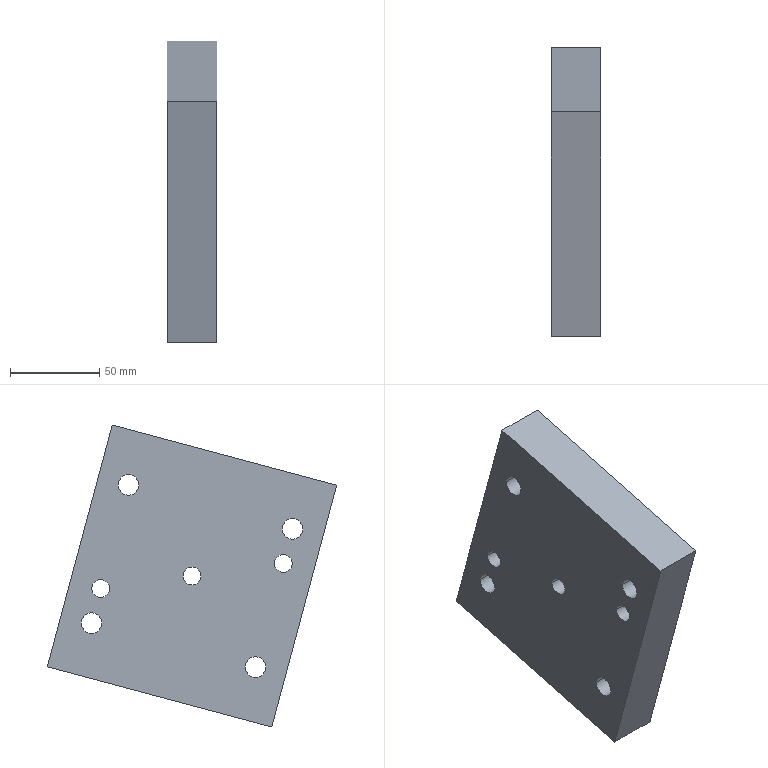Component | SolidWorks | EndFacePressurePlate-1 | 1 solid | 20 faces | box 27.78 x 161.81 x 168.88 mm | volume 487328 mm3 | cylinder 14 | plane 6 | commonest cylinder face diameters 11.57 x8 10 x6
build123d program:
from build123d import *

# Parameters (mm, degrees)
SKETCH1_R           = 5
SKETCH1_R_2         = 5.785
BOSS_EXTRUDE1_DEPTH = 27.778


with BuildPart() as part:
    # Sketch1 → Boss-Extrude1 (new body)
    with BuildSketch(Plane.XY.offset(27.778)):
        Polygon((197.028, -109.036), (71.458, -142.682), (107.693, -277.912), (233.263, -244.265), align=None)
        with Locations(Location((152.36, -193.474, 0), (0, 0, 180))):
            Circle(SKETCH1_R, mode=Mode.SUBTRACT)
        with Locations(Location((101.303, -186.449, 0), (0, 0, 180))):
            Circle(SKETCH1_R, mode=Mode.SUBTRACT)
        with Locations(Location((96.126, -167.131, 0), (0, 0, 180))):
            Circle(SKETCH1_R_2, mode=Mode.SUBTRACT)
        with Locations(Location((208.595, -219.817, 0), (0, 0, 180))):
            Circle(SKETCH1_R_2, mode=Mode.SUBTRACT)
        with Locations(Location((116.832, -244.405, 0), (0, 0, 180))):
            Circle(SKETCH1_R_2, mode=Mode.SUBTRACT)
        with Locations(Location((187.889, -142.543, 0), (0, 0, 180))):
            Circle(SKETCH1_R_2, mode=Mode.SUBTRACT)
        with Locations(Location((203.418, -200.498, 0), (0, 0, 180))):
            Circle(SKETCH1_R, mode=Mode.SUBTRACT)
    extrude(amount=-BOSS_EXTRUDE1_DEPTH)


solid = part.part

# Placed as in the assembly
solid = solid.moved(Location((-252.332, 870.769, 1116.347), (90, 90, 0)))
STEP:
#1=COLOUR_RGB('',0.7922,0.8196,0.9333);
#2=FILL_AREA_STYLE_COLOUR('',#1);
#3=FILL_AREA_STYLE('',(#2));
#4=SURFACE_STYLE_FILL_AREA(#3);
#5=SURFACE_SIDE_STYLE('',(#4));
#6=SURFACE_STYLE_USAGE(.BOTH.,#5);
#7=PRESENTATION_STYLE_ASSIGNMENT((#6));
#8=CARTESIAN_POINT('',(-9.934,42.094,36.057));
#9=VERTEX_POINT('',#8);
#10=CARTESIAN_POINT('',(-9.934,42.488,36.057));
#11=VERTEX_POINT('',#10);
#12=CARTESIAN_POINT('',(-9.934,42.291,36.057));
#13=DIRECTION('',(1.,0.,0.));
#14=DIRECTION('',(0.,-1.,0.));
#15=AXIS2_PLACEMENT_3D('',#12,#13,#14);
#16=CIRCLE('',#15,0.1969);
#17=EDGE_CURVE('',#9,#11,#16,.T.);
#18=ORIENTED_EDGE('',*,*,#17,.F.);
#19=CARTESIAN_POINT('',(-8.841,42.094,36.057));
#20=VERTEX_POINT('',#19);
#21=CARTESIAN_POINT('',(-9.934,42.094,36.057));
#22=DIRECTION('',(1.,0.,0.));
#23=VECTOR('',#22,39.37);
#24=LINE('',#21,#23);
#25=EDGE_CURVE('',#9,#20,#24,.T.);
#26=ORIENTED_EDGE('',*,*,#25,.T.);
#27=CARTESIAN_POINT('',(-8.841,42.488,36.057));
#28=VERTEX_POINT('',#27);
#29=CARTESIAN_POINT('',(-8.841,42.291,36.057));
#30=DIRECTION('',(1.,0.,0.));
#31=DIRECTION('',(0.,-1.,0.));
#32=AXIS2_PLACEMENT_3D('',#29,#30,#31);
#33=CIRCLE('',#32,0.1969);
#34=EDGE_CURVE('',#20,#28,#33,.T.);
#35=ORIENTED_EDGE('',*,*,#34,.T.);
#36=CARTESIAN_POINT('',(-9.934,42.488,36.057));
#37=DIRECTION('',(1.,0.,0.));
#38=VECTOR('',#37,39.37);
#39=LINE('',#36,#38);
#40=EDGE_CURVE('',#11,#28,#39,.T.);
#41=ORIENTED_EDGE('',*,*,#40,.F.);
#42=EDGE_LOOP('',(#18,#26,#35,#41));
#43=FACE_OUTER_BOUND('',#42,.T.);
#44=CARTESIAN_POINT('',(-9.934,42.291,36.057));
#45=DIRECTION('',(1.,0.,0.));
#46=DIRECTION('',(0.,1.,0.));
#47=AXIS2_PLACEMENT_3D('',#44,#45,#46);
#48=CYLINDRICAL_SURFACE('',#47,0.1969);
#49=ADVANCED_FACE('',(#43),#48,.F.);
#50=CARTESIAN_POINT('',(-9.934,41.452,38.339));
#51=VERTEX_POINT('',#50);
#52=CARTESIAN_POINT('',(-9.934,41.907,38.339));
#53=VERTEX_POINT('',#52);
#54=CARTESIAN_POINT('',(-9.934,41.679,38.339));
#55=DIRECTION('',(1.,0.,0.));
#56=DIRECTION('',(0.,-1.,0.));
#57=AXIS2_PLACEMENT_3D('',#54,#55,#56);
#58=CIRCLE('',#57,0.2278);
#59=EDGE_CURVE('',#51,#53,#58,.T.);
#60=ORIENTED_EDGE('',*,*,#59,.F.);
#61=CARTESIAN_POINT('',(-8.841,41.452,38.339));
#62=VERTEX_POINT('',#61);
#63=CARTESIAN_POINT('',(-9.934,41.452,38.339));
#64=DIRECTION('',(1.,0.,0.));
#65=VECTOR('',#64,39.37);
#66=LINE('',#63,#65);
#67=EDGE_CURVE('',#51,#62,#66,.T.);
#68=ORIENTED_EDGE('',*,*,#67,.T.);
#69=CARTESIAN_POINT('',(-8.841,41.907,38.339));
#70=VERTEX_POINT('',#69);
#71=CARTESIAN_POINT('',(-8.841,41.679,38.339));
#72=DIRECTION('',(1.,0.,0.));
#73=DIRECTION('',(0.,-1.,0.));
#74=AXIS2_PLACEMENT_3D('',#71,#72,#73);
#75=CIRCLE('',#74,0.2278);
#76=EDGE_CURVE('',#62,#70,#75,.T.);
#77=ORIENTED_EDGE('',*,*,#76,.T.);
#78=CARTESIAN_POINT('',(-9.934,41.907,38.339));
#79=DIRECTION('',(1.,0.,0.));
#80=VECTOR('',#79,39.37);
#81=LINE('',#78,#80);
#82=EDGE_CURVE('',#53,#70,#81,.T.);
#83=ORIENTED_EDGE('',*,*,#82,.F.);
#84=EDGE_LOOP('',(#60,#68,#77,#83));
#85=FACE_OUTER_BOUND('',#84,.T.);
#86=CARTESIAN_POINT('',(-9.934,41.679,38.339));
#87=DIRECTION('',(1.,0.,0.));
#88=DIRECTION('',(0.,1.,0.));
#89=AXIS2_PLACEMENT_3D('',#86,#87,#88);
#90=CYLINDRICAL_SURFACE('',#89,0.2278);
#91=ADVANCED_FACE('',(#85),#90,.F.);
#92=CARTESIAN_POINT('',(-9.934,38.654,34.328));
#93=VERTEX_POINT('',#92);
#94=CARTESIAN_POINT('',(-9.934,39.11,34.328));
#95=VERTEX_POINT('',#94);
#96=CARTESIAN_POINT('',(-9.934,38.882,34.328));
#97=DIRECTION('',(1.,0.,0.));
#98=DIRECTION('',(0.,-1.,0.));
#99=AXIS2_PLACEMENT_3D('',#96,#97,#98);
#100=CIRCLE('',#99,0.2278);
#101=EDGE_CURVE('',#93,#95,#100,.T.);
#102=ORIENTED_EDGE('',*,*,#101,.F.);
#103=CARTESIAN_POINT('',(-8.841,38.654,34.328));
#104=VERTEX_POINT('',#103);
#105=CARTESIAN_POINT('',(-9.934,38.654,34.328));
#106=DIRECTION('',(1.,0.,0.));
#107=VECTOR('',#106,39.37);
#108=LINE('',#105,#107);
#109=EDGE_CURVE('',#93,#104,#108,.T.);
#110=ORIENTED_EDGE('',*,*,#109,.T.);
#111=CARTESIAN_POINT('',(-8.841,39.11,34.328));
#112=VERTEX_POINT('',#111);
#113=CARTESIAN_POINT('',(-8.841,38.882,34.328));
#114=DIRECTION('',(1.,0.,0.));
#115=DIRECTION('',(0.,-1.,0.));
#116=AXIS2_PLACEMENT_3D('',#113,#114,#115);
#117=CIRCLE('',#116,0.2278);
#118=EDGE_CURVE('',#104,#112,#117,.T.);
#119=ORIENTED_EDGE('',*,*,#118,.T.);
#120=CARTESIAN_POINT('',(-9.934,39.11,34.328));
#121=DIRECTION('',(1.,0.,0.));
#122=VECTOR('',#121,39.37);
#123=LINE('',#120,#122);
#124=EDGE_CURVE('',#95,#112,#123,.T.);
#125=ORIENTED_EDGE('',*,*,#124,.F.);
#126=EDGE_LOOP('',(#102,#110,#119,#125));
#127=FACE_OUTER_BOUND('',#126,.T.);
#128=CARTESIAN_POINT('',(-9.934,38.882,34.328));
#129=DIRECTION('',(1.,0.,0.));
#130=DIRECTION('',(0.,1.,0.));
#131=AXIS2_PLACEMENT_3D('',#128,#129,#130);
#132=CYLINDRICAL_SURFACE('',#131,0.2278);
#133=ADVANCED_FACE('',(#127),#132,.F.);
#134=CARTESIAN_POINT('',(-9.934,42.267,35.296));
#135=VERTEX_POINT('',#134);
#136=CARTESIAN_POINT('',(-9.934,42.722,35.296));
#137=VERTEX_POINT('',#136);
#138=CARTESIAN_POINT('',(-9.934,42.495,35.296));
#139=DIRECTION('',(1.,0.,0.));
#140=DIRECTION('',(0.,-1.,0.));
#141=AXIS2_PLACEMENT_3D('',#138,#139,#140);
#142=CIRCLE('',#141,0.2278);
#143=EDGE_CURVE('',#135,#137,#142,.T.);
#144=ORIENTED_EDGE('',*,*,#143,.F.);
#145=CARTESIAN_POINT('',(-8.841,42.267,35.296));
#146=VERTEX_POINT('',#145);
#147=CARTESIAN_POINT('',(-9.934,42.267,35.296));
#148=DIRECTION('',(1.,0.,0.));
#149=VECTOR('',#148,39.37);
#150=LINE('',#147,#149);
#151=EDGE_CURVE('',#135,#146,#150,.T.);
#152=ORIENTED_EDGE('',*,*,#151,.T.);
#153=CARTESIAN_POINT('',(-8.841,42.722,35.296));
#154=VERTEX_POINT('',#153);
#155=CARTESIAN_POINT('',(-8.841,42.495,35.296));
#156=DIRECTION('',(1.,0.,0.));
#157=DIRECTION('',(0.,-1.,0.));
#158=AXIS2_PLACEMENT_3D('',#155,#156,#157);
#159=CIRCLE('',#158,0.2278);
#160=EDGE_CURVE('',#146,#154,#159,.T.);
#161=ORIENTED_EDGE('',*,*,#160,.T.);
#162=CARTESIAN_POINT('',(-9.934,42.722,35.296));
#163=DIRECTION('',(1.,0.,0.));
#164=VECTOR('',#163,39.37);
#165=LINE('',#162,#164);
#166=EDGE_CURVE('',#137,#154,#165,.T.);
#167=ORIENTED_EDGE('',*,*,#166,.F.);
#168=EDGE_LOOP('',(#144,#152,#161,#167));
#169=FACE_OUTER_BOUND('',#168,.T.);
#170=CARTESIAN_POINT('',(-9.934,42.495,35.296));
#171=DIRECTION('',(1.,0.,0.));
#172=DIRECTION('',(0.,1.,0.));
#173=AXIS2_PLACEMENT_3D('',#170,#171,#172);
#174=CYLINDRICAL_SURFACE('',#173,0.2278);
#175=ADVANCED_FACE('',(#169),#174,.F.);
#176=CARTESIAN_POINT('',(-9.934,37.839,37.371));
#177=VERTEX_POINT('',#176);
#178=CARTESIAN_POINT('',(-9.934,38.294,37.371));
#179=VERTEX_POINT('',#178);
#180=CARTESIAN_POINT('',(-9.934,38.067,37.371));
#181=DIRECTION('',(1.,0.,0.));
#182=DIRECTION('',(0.,-1.,0.));
#183=AXIS2_PLACEMENT_3D('',#180,#181,#182);
#184=CIRCLE('',#183,0.2278);
#185=EDGE_CURVE('',#177,#179,#184,.T.);
#186=ORIENTED_EDGE('',*,*,#185,.F.);
#187=CARTESIAN_POINT('',(-8.841,37.839,37.371));
#188=VERTEX_POINT('',#187);
#189=CARTESIAN_POINT('',(-9.934,37.839,37.371));
#190=DIRECTION('',(1.,0.,0.));
#191=VECTOR('',#190,39.37);
#192=LINE('',#189,#191);
#193=EDGE_CURVE('',#177,#188,#192,.T.);
#194=ORIENTED_EDGE('',*,*,#193,.T.);
#195=CARTESIAN_POINT('',(-8.841,38.294,37.371));
#196=VERTEX_POINT('',#195);
#197=CARTESIAN_POINT('',(-8.841,38.067,37.371));
#198=DIRECTION('',(1.,0.,0.));
#199=DIRECTION('',(0.,-1.,0.));
#200=AXIS2_PLACEMENT_3D('',#197,#198,#199);
#201=CIRCLE('',#200,0.2278);
#202=EDGE_CURVE('',#188,#196,#201,.T.);
#203=ORIENTED_EDGE('',*,*,#202,.T.);
#204=CARTESIAN_POINT('',(-9.934,38.294,37.371));
#205=DIRECTION('',(1.,0.,0.));
#206=VECTOR('',#205,39.37);
#207=LINE('',#204,#206);
#208=EDGE_CURVE('',#179,#196,#207,.T.);
#209=ORIENTED_EDGE('',*,*,#208,.F.);
#210=EDGE_LOOP('',(#186,#194,#203,#209));
#211=FACE_OUTER_BOUND('',#210,.T.);
#212=CARTESIAN_POINT('',(-9.934,38.067,37.371));
#213=DIRECTION('',(1.,0.,0.));
#214=DIRECTION('',(0.,1.,0.));
#215=AXIS2_PLACEMENT_3D('',#212,#213,#214);
#216=CYLINDRICAL_SURFACE('',#215,0.2278);
#217=ADVANCED_FACE('',(#211),#216,.F.);
#218=CARTESIAN_POINT('',(-9.934,38.074,36.61));
#219=VERTEX_POINT('',#218);
#220=CARTESIAN_POINT('',(-9.934,38.467,36.61));
#221=VERTEX_POINT('',#220);
#222=CARTESIAN_POINT('',(-9.934,38.271,36.61));
#223=DIRECTION('',(1.,0.,0.));
#224=DIRECTION('',(0.,-1.,0.));
#225=AXIS2_PLACEMENT_3D('',#222,#223,#224);
#226=CIRCLE('',#225,0.1969);
#227=EDGE_CURVE('',#219,#221,#226,.T.);
#228=ORIENTED_EDGE('',*,*,#227,.F.);
#229=CARTESIAN_POINT('',(-8.841,38.074,36.61));
#230=VERTEX_POINT('',#229);
#231=CARTESIAN_POINT('',(-9.934,38.074,36.61));
#232=DIRECTION('',(1.,0.,0.));
#233=VECTOR('',#232,39.37);
#234=LINE('',#231,#233);
#235=EDGE_CURVE('',#219,#230,#234,.T.);
#236=ORIENTED_EDGE('',*,*,#235,.T.);
#237=CARTESIAN_POINT('',(-8.841,38.467,36.61));
#238=VERTEX_POINT('',#237);
#239=CARTESIAN_POINT('',(-8.841,38.271,36.61));
#240=DIRECTION('',(1.,0.,0.));
#241=DIRECTION('',(0.,-1.,0.));
#242=AXIS2_PLACEMENT_3D('',#239,#240,#241);
#243=CIRCLE('',#242,0.1969);
#244=EDGE_CURVE('',#230,#238,#243,.T.);
#245=ORIENTED_EDGE('',*,*,#244,.T.);
#246=CARTESIAN_POINT('',(-9.934,38.467,36.61));
#247=DIRECTION('',(1.,0.,0.));
#248=VECTOR('',#247,39.37);
#249=LINE('',#246,#248);
#250=EDGE_CURVE('',#221,#238,#249,.T.);
#251=ORIENTED_EDGE('',*,*,#250,.F.);
#252=EDGE_LOOP('',(#228,#236,#245,#251));
#253=FACE_OUTER_BOUND('',#252,.T.);
#254=CARTESIAN_POINT('',(-9.934,38.271,36.61));
#255=DIRECTION('',(1.,0.,0.));
#256=DIRECTION('',(0.,1.,0.));
#257=AXIS2_PLACEMENT_3D('',#254,#255,#256);
#258=CYLINDRICAL_SURFACE('',#257,0.1969);
#259=ADVANCED_FACE('',(#253),#258,.F.);
#260=CARTESIAN_POINT('',(-9.934,40.084,36.334));
#261=VERTEX_POINT('',#260);
#262=CARTESIAN_POINT('',(-9.934,40.478,36.334));
#263=VERTEX_POINT('',#262);
#264=CARTESIAN_POINT('',(-9.934,40.281,36.334));
#265=DIRECTION('',(1.,0.,0.));
#266=DIRECTION('',(0.,-1.,0.));
#267=AXIS2_PLACEMENT_3D('',#264,#265,#266);
#268=CIRCLE('',#267,0.1969);
#269=EDGE_CURVE('',#261,#263,#268,.T.);
#270=ORIENTED_EDGE('',*,*,#269,.F.);
#271=CARTESIAN_POINT('',(-8.841,40.084,36.334));
#272=VERTEX_POINT('',#271);
#273=CARTESIAN_POINT('',(-9.934,40.084,36.334));
#274=DIRECTION('',(1.,0.,0.));
#275=VECTOR('',#274,39.37);
#276=LINE('',#273,#275);
#277=EDGE_CURVE('',#261,#272,#276,.T.);
#278=ORIENTED_EDGE('',*,*,#277,.T.);
#279=CARTESIAN_POINT('',(-8.841,40.478,36.334));
#280=VERTEX_POINT('',#279);
#281=CARTESIAN_POINT('',(-8.841,40.281,36.334));
#282=DIRECTION('',(1.,0.,0.));
#283=DIRECTION('',(0.,-1.,0.));
#284=AXIS2_PLACEMENT_3D('',#281,#282,#283);
#285=CIRCLE('',#284,0.1969);
#286=EDGE_CURVE('',#272,#280,#285,.T.);
#287=ORIENTED_EDGE('',*,*,#286,.T.);
#288=CARTESIAN_POINT('',(-9.934,40.478,36.334));
#289=DIRECTION('',(1.,0.,0.));
#290=VECTOR('',#289,39.37);
#291=LINE('',#288,#290);
#292=EDGE_CURVE('',#263,#280,#291,.T.);
#293=ORIENTED_EDGE('',*,*,#292,.F.);
#294=EDGE_LOOP('',(#270,#278,#287,#293));
#295=FACE_OUTER_BOUND('',#294,.T.);
#296=CARTESIAN_POINT('',(-9.934,40.281,36.334));
#297=DIRECTION('',(1.,0.,0.));
#298=DIRECTION('',(0.,1.,0.));
#299=AXIS2_PLACEMENT_3D('',#296,#297,#298);
#300=CYLINDRICAL_SURFACE('',#299,0.1969);
#301=ADVANCED_FACE('',(#295),#300,.F.);
#302=CARTESIAN_POINT('',(-8.841,43.466,34.334));
#303=VERTEX_POINT('',#302);
#304=CARTESIAN_POINT('',(-8.841,42.039,39.658));
#305=VERTEX_POINT('',#304);
#306=CARTESIAN_POINT('',(-8.841,43.466,34.334));
#307=DIRECTION('',(0.,-0.2588,0.9659));
#308=VECTOR('',#307,39.37);
#309=LINE('',#306,#308);
#310=EDGE_CURVE('',#303,#305,#309,.T.);
#311=ORIENTED_EDGE('',*,*,#310,.F.);
#312=CARTESIAN_POINT('',(-9.934,43.466,34.334));
#313=VERTEX_POINT('',#312);
#314=CARTESIAN_POINT('',(-9.934,43.466,34.334));
#315=DIRECTION('',(1.,0.,0.));
#316=VECTOR('',#315,39.37);
#317=LINE('',#314,#316);
#318=EDGE_CURVE('',#313,#303,#317,.T.);
#319=ORIENTED_EDGE('',*,*,#318,.F.);
#320=CARTESIAN_POINT('',(-9.934,42.039,39.658));
#321=VERTEX_POINT('',#320);
#322=CARTESIAN_POINT('',(-9.934,43.466,34.334));
#323=DIRECTION('',(0.,-0.2588,0.9659));
#324=VECTOR('',#323,39.37);
#325=LINE('',#322,#324);
#326=EDGE_CURVE('',#313,#321,#325,.T.);
#327=ORIENTED_EDGE('',*,*,#326,.T.);
#328=CARTESIAN_POINT('',(-9.934,42.039,39.658));
#329=DIRECTION('',(1.,0.,0.));
#330=VECTOR('',#329,39.37);
#331=LINE('',#328,#330);
#332=EDGE_CURVE('',#321,#305,#331,.T.);
#333=ORIENTED_EDGE('',*,*,#332,.T.);
#334=EDGE_LOOP('',(#311,#319,#327,#333));
#335=FACE_OUTER_BOUND('',#334,.T.);
#336=CARTESIAN_POINT('',(-9.934,43.466,34.334));
#337=DIRECTION('',(0.,0.9659,0.2588));
#338=DIRECTION('',(0.,-0.2588,0.9659));
#339=AXIS2_PLACEMENT_3D('',#336,#337,#338);
#340=PLANE('',#339);
#341=ADVANCED_FACE('',(#335),#340,.T.);
#342=CARTESIAN_POINT('',(-8.841,38.522,33.009));
#343=VERTEX_POINT('',#342);
#344=CARTESIAN_POINT('',(-8.841,38.522,33.009));
#345=DIRECTION('',(0.,0.9659,0.2588));
#346=VECTOR('',#345,39.37);
#347=LINE('',#344,#346);
#348=EDGE_CURVE('',#343,#303,#347,.T.);
#349=ORIENTED_EDGE('',*,*,#348,.F.);
#350=CARTESIAN_POINT('',(-9.934,38.522,33.009));
#351=VERTEX_POINT('',#350);
#352=CARTESIAN_POINT('',(-9.934,38.522,33.009));
#353=DIRECTION('',(1.,0.,0.));
#354=VECTOR('',#353,39.37);
#355=LINE('',#352,#354);
#356=EDGE_CURVE('',#351,#343,#355,.T.);
#357=ORIENTED_EDGE('',*,*,#356,.F.);
#358=CARTESIAN_POINT('',(-9.934,38.522,33.009));
#359=DIRECTION('',(0.,0.9659,0.2588));
#360=VECTOR('',#359,39.37);
#361=LINE('',#358,#360);
#362=EDGE_CURVE('',#351,#313,#361,.T.);
#363=ORIENTED_EDGE('',*,*,#362,.T.);
#364=ORIENTED_EDGE('',*,*,#318,.T.);
#365=EDGE_LOOP('',(#349,#357,#363,#364));
#366=FACE_OUTER_BOUND('',#365,.T.);
#367=CARTESIAN_POINT('',(-9.934,38.522,33.009));
#368=DIRECTION('',(0.,0.2588,-0.9659));
#369=DIRECTION('',(0.,0.9659,0.2588));
#370=AXIS2_PLACEMENT_3D('',#367,#368,#369);
#371=PLANE('',#370);
#372=ADVANCED_FACE('',(#366),#371,.T.);
#373=CARTESIAN_POINT('',(-8.841,37.096,38.333));
#374=VERTEX_POINT('',#373);
#375=CARTESIAN_POINT('',(-8.841,37.096,38.333));
#376=DIRECTION('',(0.,0.2588,-0.9659));
#377=VECTOR('',#376,39.37);
#378=LINE('',#375,#377);
#379=EDGE_CURVE('',#374,#343,#378,.T.);
#380=ORIENTED_EDGE('',*,*,#379,.F.);
#381=CARTESIAN_POINT('',(-9.934,37.096,38.333));
#382=VERTEX_POINT('',#381);
#383=CARTESIAN_POINT('',(-9.934,37.096,38.333));
#384=DIRECTION('',(1.,0.,0.));
#385=VECTOR('',#384,39.37);
#386=LINE('',#383,#385);
#387=EDGE_CURVE('',#382,#374,#386,.T.);
#388=ORIENTED_EDGE('',*,*,#387,.F.);
#389=CARTESIAN_POINT('',(-9.934,37.096,38.333));
#390=DIRECTION('',(0.,0.2588,-0.9659));
#391=VECTOR('',#390,39.37);
#392=LINE('',#389,#391);
#393=EDGE_CURVE('',#382,#351,#392,.T.);
#394=ORIENTED_EDGE('',*,*,#393,.T.);
#395=ORIENTED_EDGE('',*,*,#356,.T.);
#396=EDGE_LOOP('',(#380,#388,#394,#395));
#397=FACE_OUTER_BOUND('',#396,.T.);
#398=CARTESIAN_POINT('',(-9.934,37.096,38.333));
#399=DIRECTION('',(0.,-0.9659,-0.2588));
#400=DIRECTION('',(0.,0.2588,-0.9659));
#401=AXIS2_PLACEMENT_3D('',#398,#399,#400);
#402=PLANE('',#401);
#403=ADVANCED_FACE('',(#397),#402,.T.);
#404=CARTESIAN_POINT('',(-8.841,42.039,39.658));
#405=DIRECTION('',(0.,-0.9659,-0.2588));
#406=VECTOR('',#405,39.37);
#407=LINE('',#404,#406);
#408=EDGE_CURVE('',#305,#374,#407,.T.);
#409=ORIENTED_EDGE('',*,*,#408,.F.);
#410=ORIENTED_EDGE('',*,*,#332,.F.);
#411=CARTESIAN_POINT('',(-9.934,42.039,39.658));
#412=DIRECTION('',(0.,-0.9659,-0.2588));
#413=VECTOR('',#412,39.37);
#414=LINE('',#411,#413);
#415=EDGE_CURVE('',#321,#382,#414,.T.);
#416=ORIENTED_EDGE('',*,*,#415,.T.);
#417=ORIENTED_EDGE('',*,*,#387,.T.);
#418=EDGE_LOOP('',(#409,#410,#416,#417));
#419=FACE_OUTER_BOUND('',#418,.T.);
#420=CARTESIAN_POINT('',(-9.934,42.039,39.658));
#421=DIRECTION('',(0.,-0.2588,0.9659));
#422=DIRECTION('',(0.,-0.9659,-0.2588));
#423=AXIS2_PLACEMENT_3D('',#420,#421,#422);
#424=PLANE('',#423);
#425=ADVANCED_FACE('',(#419),#424,.T.);
#426=CARTESIAN_POINT('',(-9.934,42.291,36.057));
#427=DIRECTION('',(1.,0.,0.));
#428=DIRECTION('',(0.,-1.,0.));
#429=AXIS2_PLACEMENT_3D('',#426,#427,#428);
#430=CIRCLE('',#429,0.1969);
#431=EDGE_CURVE('',#11,#9,#430,.T.);
#432=ORIENTED_EDGE('',*,*,#431,.T.);
#433=ORIENTED_EDGE('',*,*,#17,.T.);
#434=EDGE_LOOP('',(#432,#433));
#435=FACE_BOUND('',#434,.T.);
#436=CARTESIAN_POINT('',(-9.934,41.679,38.339));
#437=DIRECTION('',(1.,0.,0.));
#438=DIRECTION('',(0.,-1.,0.));
#439=AXIS2_PLACEMENT_3D('',#436,#437,#438);
#440=CIRCLE('',#439,0.2278);
#441=EDGE_CURVE('',#53,#51,#440,.T.);
#442=ORIENTED_EDGE('',*,*,#441,.T.);
#443=ORIENTED_EDGE('',*,*,#59,.T.);
#444=EDGE_LOOP('',(#442,#443));
#445=FACE_BOUND('',#444,.T.);
#446=CARTESIAN_POINT('',(-9.934,38.882,34.328));
#447=DIRECTION('',(1.,0.,0.));
#448=DIRECTION('',(0.,-1.,0.));
#449=AXIS2_PLACEMENT_3D('',#446,#447,#448);
#450=CIRCLE('',#449,0.2278);
#451=EDGE_CURVE('',#95,#93,#450,.T.);
#452=ORIENTED_EDGE('',*,*,#451,.T.);
#453=ORIENTED_EDGE('',*,*,#101,.T.);
#454=EDGE_LOOP('',(#452,#453));
#455=FACE_BOUND('',#454,.T.);
#456=CARTESIAN_POINT('',(-9.934,42.495,35.296));
#457=DIRECTION('',(1.,0.,0.));
#458=DIRECTION('',(0.,-1.,0.));
#459=AXIS2_PLACEMENT_3D('',#456,#457,#458);
#460=CIRCLE('',#459,0.2278);
#461=EDGE_CURVE('',#137,#135,#460,.T.);
#462=ORIENTED_EDGE('',*,*,#461,.T.);
#463=ORIENTED_EDGE('',*,*,#143,.T.);
#464=EDGE_LOOP('',(#462,#463));
#465=FACE_BOUND('',#464,.T.);
#466=CARTESIAN_POINT('',(-9.934,38.067,37.371));
#467=DIRECTION('',(1.,0.,0.));
#468=DIRECTION('',(0.,-1.,0.));
#469=AXIS2_PLACEMENT_3D('',#466,#467,#468);
#470=CIRCLE('',#469,0.2278);
#471=EDGE_CURVE('',#179,#177,#470,.T.);
#472=ORIENTED_EDGE('',*,*,#471,.T.);
#473=ORIENTED_EDGE('',*,*,#185,.T.);
#474=EDGE_LOOP('',(#472,#473));
#475=FACE_BOUND('',#474,.T.);
#476=CARTESIAN_POINT('',(-9.934,38.271,36.61));
#477=DIRECTION('',(1.,0.,0.));
#478=DIRECTION('',(0.,-1.,0.));
#479=AXIS2_PLACEMENT_3D('',#476,#477,#478);
#480=CIRCLE('',#479,0.1969);
#481=EDGE_CURVE('',#221,#219,#480,.T.);
#482=ORIENTED_EDGE('',*,*,#481,.T.);
#483=ORIENTED_EDGE('',*,*,#227,.T.);
#484=EDGE_LOOP('',(#482,#483));
#485=FACE_BOUND('',#484,.T.);
#486=CARTESIAN_POINT('',(-9.934,40.281,36.334));
#487=DIRECTION('',(1.,0.,0.));
#488=DIRECTION('',(0.,-1.,0.));
#489=AXIS2_PLACEMENT_3D('',#486,#487,#488);
#490=CIRCLE('',#489,0.1969);
#491=EDGE_CURVE('',#263,#261,#490,.T.);
#492=ORIENTED_EDGE('',*,*,#491,.T.);
#493=ORIENTED_EDGE('',*,*,#269,.T.);
#494=EDGE_LOOP('',(#492,#493));
#495=FACE_BOUND('',#494,.T.);
#496=ORIENTED_EDGE('',*,*,#326,.F.);
#497=ORIENTED_EDGE('',*,*,#362,.F.);
#498=ORIENTED_EDGE('',*,*,#393,.F.);
#499=ORIENTED_EDGE('',*,*,#415,.F.);
#500=EDGE_LOOP('',(#496,#497,#498,#499));
#501=FACE_OUTER_BOUND('',#500,.T.);
#502=CARTESIAN_POINT('',(-9.934,34.282,43.951));
#503=DIRECTION('',(1.,0.,0.));
#504=DIRECTION('',(0.,1.,0.));
#505=AXIS2_PLACEMENT_3D('',#502,#503,#504);
#506=PLANE('',#505);
#507=ADVANCED_FACE('',(#435,#445,#455,#465,#475,#485,#495,#501),#506,.F.);
#508=CARTESIAN_POINT('',(-8.841,42.291,36.057));
#509=DIRECTION('',(1.,0.,0.));
#510=DIRECTION('',(0.,-1.,0.));
#511=AXIS2_PLACEMENT_3D('',#508,#509,#510);
#512=CIRCLE('',#511,0.1969);
#513=EDGE_CURVE('',#28,#20,#512,.T.);
#514=ORIENTED_EDGE('',*,*,#513,.F.);
#515=ORIENTED_EDGE('',*,*,#34,.F.);
#516=EDGE_LOOP('',(#514,#515));
#517=FACE_BOUND('',#516,.T.);
#518=CARTESIAN_POINT('',(-8.841,41.679,38.339));
#519=DIRECTION('',(1.,0.,0.));
#520=DIRECTION('',(0.,-1.,0.));
#521=AXIS2_PLACEMENT_3D('',#518,#519,#520);
#522=CIRCLE('',#521,0.2278);
#523=EDGE_CURVE('',#70,#62,#522,.T.);
#524=ORIENTED_EDGE('',*,*,#523,.F.);
#525=ORIENTED_EDGE('',*,*,#76,.F.);
#526=EDGE_LOOP('',(#524,#525));
#527=FACE_BOUND('',#526,.T.);
#528=CARTESIAN_POINT('',(-8.841,38.882,34.328));
#529=DIRECTION('',(1.,0.,0.));
#530=DIRECTION('',(0.,-1.,0.));
#531=AXIS2_PLACEMENT_3D('',#528,#529,#530);
#532=CIRCLE('',#531,0.2278);
#533=EDGE_CURVE('',#112,#104,#532,.T.);
#534=ORIENTED_EDGE('',*,*,#533,.F.);
#535=ORIENTED_EDGE('',*,*,#118,.F.);
#536=EDGE_LOOP('',(#534,#535));
#537=FACE_BOUND('',#536,.T.);
#538=CARTESIAN_POINT('',(-8.841,42.495,35.296));
#539=DIRECTION('',(1.,0.,0.));
#540=DIRECTION('',(0.,-1.,0.));
#541=AXIS2_PLACEMENT_3D('',#538,#539,#540);
#542=CIRCLE('',#541,0.2278);
#543=EDGE_CURVE('',#154,#146,#542,.T.);
#544=ORIENTED_EDGE('',*,*,#543,.F.);
#545=ORIENTED_EDGE('',*,*,#160,.F.);
#546=EDGE_LOOP('',(#544,#545));
#547=FACE_BOUND('',#546,.T.);
#548=CARTESIAN_POINT('',(-8.841,38.067,37.371));
#549=DIRECTION('',(1.,0.,0.));
#550=DIRECTION('',(0.,-1.,0.));
#551=AXIS2_PLACEMENT_3D('',#548,#549,#550);
#552=CIRCLE('',#551,0.2278);
#553=EDGE_CURVE('',#196,#188,#552,.T.);
#554=ORIENTED_EDGE('',*,*,#553,.F.);
#555=ORIENTED_EDGE('',*,*,#202,.F.);
#556=EDGE_LOOP('',(#554,#555));
#557=FACE_BOUND('',#556,.T.);
#558=CARTESIAN_POINT('',(-8.841,38.271,36.61));
#559=DIRECTION('',(1.,0.,0.));
#560=DIRECTION('',(0.,-1.,0.));
#561=AXIS2_PLACEMENT_3D('',#558,#559,#560);
#562=CIRCLE('',#561,0.1969);
#563=EDGE_CURVE('',#238,#230,#562,.T.);
#564=ORIENTED_EDGE('',*,*,#563,.F.);
#565=ORIENTED_EDGE('',*,*,#244,.F.);
#566=EDGE_LOOP('',(#564,#565));
#567=FACE_BOUND('',#566,.T.);
#568=CARTESIAN_POINT('',(-8.841,40.281,36.334));
#569=DIRECTION('',(1.,0.,0.));
#570=DIRECTION('',(0.,-1.,0.));
#571=AXIS2_PLACEMENT_3D('',#568,#569,#570);
#572=CIRCLE('',#571,0.1969);
#573=EDGE_CURVE('',#280,#272,#572,.T.);
#574=ORIENTED_EDGE('',*,*,#573,.F.);
#575=ORIENTED_EDGE('',*,*,#286,.F.);
#576=EDGE_LOOP('',(#574,#575));
#577=FACE_BOUND('',#576,.T.);
#578=ORIENTED_EDGE('',*,*,#310,.T.);
#579=ORIENTED_EDGE('',*,*,#408,.T.);
#580=ORIENTED_EDGE('',*,*,#379,.T.);
#581=ORIENTED_EDGE('',*,*,#348,.T.);
#582=EDGE_LOOP('',(#578,#579,#580,#581));
#583=FACE_OUTER_BOUND('',#582,.T.);
#584=CARTESIAN_POINT('',(-8.841,34.282,43.951));
#585=DIRECTION('',(1.,0.,0.));
#586=DIRECTION('',(0.,1.,0.));
#587=AXIS2_PLACEMENT_3D('',#584,#585,#586);
#588=PLANE('',#587);
#589=ADVANCED_FACE('',(#517,#527,#537,#547,#557,#567,#577,#583),#588,.T.);
#590=ORIENTED_EDGE('',*,*,#277,.F.);
#591=ORIENTED_EDGE('',*,*,#491,.F.);
#592=ORIENTED_EDGE('',*,*,#292,.T.);
#593=ORIENTED_EDGE('',*,*,#573,.T.);
#594=EDGE_LOOP('',(#590,#591,#592,#593));
#595=FACE_OUTER_BOUND('',#594,.T.);
#596=CARTESIAN_POINT('',(-9.934,40.281,36.334));
#597=DIRECTION('',(1.,0.,0.));
#598=DIRECTION('',(0.,1.,0.));
#599=AXIS2_PLACEMENT_3D('',#596,#597,#598);
#600=CYLINDRICAL_SURFACE('',#599,0.1969);
#601=ADVANCED_FACE('',(#595),#600,.F.);
#602=ORIENTED_EDGE('',*,*,#235,.F.);
#603=ORIENTED_EDGE('',*,*,#481,.F.);
#604=ORIENTED_EDGE('',*,*,#250,.T.);
#605=ORIENTED_EDGE('',*,*,#563,.T.);
#606=EDGE_LOOP('',(#602,#603,#604,#605));
#607=FACE_OUTER_BOUND('',#606,.T.);
#608=CARTESIAN_POINT('',(-9.934,38.271,36.61));
#609=DIRECTION('',(1.,0.,0.));
#610=DIRECTION('',(0.,1.,0.));
#611=AXIS2_PLACEMENT_3D('',#608,#609,#610);
#612=CYLINDRICAL_SURFACE('',#611,0.1969);
#613=ADVANCED_FACE('',(#607),#612,.F.);
#614=ORIENTED_EDGE('',*,*,#193,.F.);
#615=ORIENTED_EDGE('',*,*,#471,.F.);
#616=ORIENTED_EDGE('',*,*,#208,.T.);
#617=ORIENTED_EDGE('',*,*,#553,.T.);
#618=EDGE_LOOP('',(#614,#615,#616,#617));
#619=FACE_OUTER_BOUND('',#618,.T.);
#620=CARTESIAN_POINT('',(-9.934,38.067,37.371));
#621=DIRECTION('',(1.,0.,0.));
#622=DIRECTION('',(0.,1.,0.));
#623=AXIS2_PLACEMENT_3D('',#620,#621,#622);
#624=CYLINDRICAL_SURFACE('',#623,0.2278);
#625=ADVANCED_FACE('',(#619),#624,.F.);
#626=ORIENTED_EDGE('',*,*,#151,.F.);
#627=ORIENTED_EDGE('',*,*,#461,.F.);
#628=ORIENTED_EDGE('',*,*,#166,.T.);
#629=ORIENTED_EDGE('',*,*,#543,.T.);
#630=EDGE_LOOP('',(#626,#627,#628,#629));
#631=FACE_OUTER_BOUND('',#630,.T.);
#632=CARTESIAN_POINT('',(-9.934,42.495,35.296));
#633=DIRECTION('',(1.,0.,0.));
#634=DIRECTION('',(0.,1.,0.));
#635=AXIS2_PLACEMENT_3D('',#632,#633,#634);
#636=CYLINDRICAL_SURFACE('',#635,0.2278);
#637=ADVANCED_FACE('',(#631),#636,.F.);
#638=ORIENTED_EDGE('',*,*,#109,.F.);
#639=ORIENTED_EDGE('',*,*,#451,.F.);
#640=ORIENTED_EDGE('',*,*,#124,.T.);
#641=ORIENTED_EDGE('',*,*,#533,.T.);
#642=EDGE_LOOP('',(#638,#639,#640,#641));
#643=FACE_OUTER_BOUND('',#642,.T.);
#644=CARTESIAN_POINT('',(-9.934,38.882,34.328));
#645=DIRECTION('',(1.,0.,0.));
#646=DIRECTION('',(0.,1.,0.));
#647=AXIS2_PLACEMENT_3D('',#644,#645,#646);
#648=CYLINDRICAL_SURFACE('',#647,0.2278);
#649=ADVANCED_FACE('',(#643),#648,.F.);
#650=ORIENTED_EDGE('',*,*,#67,.F.);
#651=ORIENTED_EDGE('',*,*,#441,.F.);
#652=ORIENTED_EDGE('',*,*,#82,.T.);
#653=ORIENTED_EDGE('',*,*,#523,.T.);
#654=EDGE_LOOP('',(#650,#651,#652,#653));
#655=FACE_OUTER_BOUND('',#654,.T.);
#656=CARTESIAN_POINT('',(-9.934,41.679,38.339));
#657=DIRECTION('',(1.,0.,0.));
#658=DIRECTION('',(0.,1.,0.));
#659=AXIS2_PLACEMENT_3D('',#656,#657,#658);
#660=CYLINDRICAL_SURFACE('',#659,0.2278);
#661=ADVANCED_FACE('',(#655),#660,.F.);
#662=ORIENTED_EDGE('',*,*,#25,.F.);
#663=ORIENTED_EDGE('',*,*,#431,.F.);
#664=ORIENTED_EDGE('',*,*,#40,.T.);
#665=ORIENTED_EDGE('',*,*,#513,.T.);
#666=EDGE_LOOP('',(#662,#663,#664,#665));
#667=FACE_OUTER_BOUND('',#666,.T.);
#668=CARTESIAN_POINT('',(-9.934,42.291,36.057));
#669=DIRECTION('',(1.,0.,0.));
#670=DIRECTION('',(0.,1.,0.));
#671=AXIS2_PLACEMENT_3D('',#668,#669,#670);
#672=CYLINDRICAL_SURFACE('',#671,0.1969);
#673=ADVANCED_FACE('',(#667),#672,.F.);
#674=CLOSED_SHELL('',(#49,#91,#133,#175,#217,#259,#301,#341,#372,#403,#425,#507,#589,#601,#613,#625,#637,#649,#661,#673));
#675=MANIFOLD_SOLID_BREP('',#674);
#676=STYLED_ITEM('',(#7),#675);
#677=PRESENTATION_LAYER_ASSIGNMENT('','',(#676));
#678=CARTESIAN_POINT('',(0.,0.,0.));
#679=DIRECTION('',(0.,0.,1.));
#680=DIRECTION('',(1.,0.,0.));
#681=AXIS2_PLACEMENT_3D('',#678,#679,#680);
#682=(LENGTH_UNIT()NAMED_UNIT(*)SI_UNIT($,.METRE.));
#683=LENGTH_MEASURE_WITH_UNIT(LENGTH_MEASURE(0.0254),#682);
#684=DIMENSIONAL_EXPONENTS(1.,0.,0.,0.,0.,0.,0.);
#685=(CONVERSION_BASED_UNIT('',#683)LENGTH_UNIT()NAMED_UNIT(#684));
#686=UNCERTAINTY_MEASURE_WITH_UNIT(LENGTH_MEASURE(0.00001),#685,'','');
#687=(NAMED_UNIT(*)PLANE_ANGLE_UNIT()SI_UNIT($,.RADIAN.));
#688=(NAMED_UNIT(*)SI_UNIT($,.STERADIAN.)SOLID_ANGLE_UNIT());
#689=(GEOMETRIC_REPRESENTATION_CONTEXT(3)GLOBAL_UNCERTAINTY_ASSIGNED_CONTEXT((#686))GLOBAL_UNIT_ASSIGNED_CONTEXT((#685,#687,#688))REPRESENTATION_CONTEXT('',''));
#690=ADVANCED_BREP_SHAPE_REPRESENTATION('',(#675,#681),#689);
#691=(LENGTH_UNIT()NAMED_UNIT(*)SI_UNIT($,.METRE.));
#692=LENGTH_MEASURE_WITH_UNIT(LENGTH_MEASURE(0.0254),#691);
#693=DIMENSIONAL_EXPONENTS(1.,0.,0.,0.,0.,0.,0.);
#694=(CONVERSION_BASED_UNIT('',#692)LENGTH_UNIT()NAMED_UNIT(#693));
#695=UNCERTAINTY_MEASURE_WITH_UNIT(LENGTH_MEASURE(0.00001),#694,'','');
#696=(NAMED_UNIT(*)PLANE_ANGLE_UNIT()SI_UNIT($,.RADIAN.));
#697=(NAMED_UNIT(*)SI_UNIT($,.STERADIAN.)SOLID_ANGLE_UNIT());
#698=(GEOMETRIC_REPRESENTATION_CONTEXT(3)GLOBAL_UNCERTAINTY_ASSIGNED_CONTEXT((#695))GLOBAL_UNIT_ASSIGNED_CONTEXT((#694,#696,#697))REPRESENTATION_CONTEXT('',''));
#699=MECHANICAL_DESIGN_GEOMETRIC_PRESENTATION_REPRESENTATION('',(#676),#698);